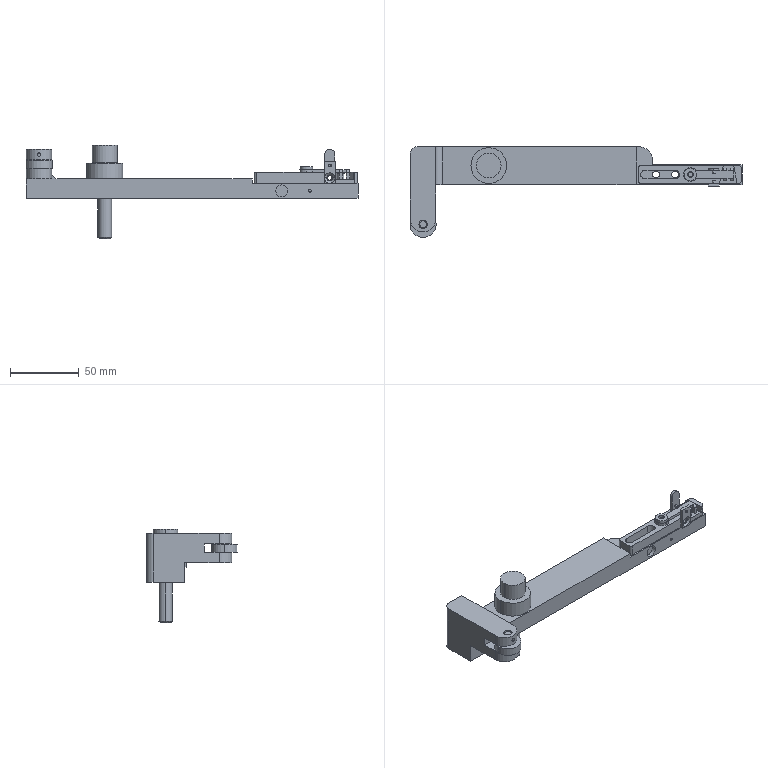Assembly | SolidWorks | mm | 13 component files | 13 solids | 202 faces | box 241.25 x 66 x 68 mm | volume 117753 mm3 | plane 98 | cylinder 82 | cone 22 | commonest cylinder face diameters 2 x10 5 x10 6 x8 4 x8 10 x7 8 x4 16 x4 12 x4
Bill of materials:
Bearing626z | 1 |  | Thick flat annular disc (ring) with a central through-hole; plain cylindrical outer face and flat parallel faces.
BSH3-02-05SmallWheel | 1 |  | Short solid cylinder, about as long as it is wide, with a chamfer on both end edges.
BSH3-02-06SpringRetainer | 1 |  | Rectangular flat plate with a small round through-hole near one end and a larger through-hole near the other end that has a conical countersink on one face.
BSH3-02-07Pin | 2 |  | Solid cylindrical pin, roughly twice as long as its diameter, with a chamfer on both ends.
BSH3-02-08BendingPlate | 1 |  | Flat bar-like bent part: an elongated strip ending in a ring-shaped eye with a round hole at one end; an upright tab with a rounded top and a small hole rising from the strip; and at the other end, legs/tabs bent down to form a U-shaped or channel-like clip section.
BSH3-02-09Gasket | 1 |  | Flanged bushing: a larger-diameter cylindrical flange plus a smaller-diameter cylindrical spigot on one side, with a straight central through-bore.
BSH3-02-10FeedBlock2 | 1 |  | Elongated rectangular bar with rounded corners. It has a long through slot with rounded ends, a small vertical through-hole, a cross hole through the side, and a stepped end region with a notch/slot cut across it.
BSH3-03-01Lever | 1 |  | Long arm/lever-like bar. At one end is a forked clevis with two parallel lugs, each with a small hole. Partway along is a raised cylindrical boss with a large bore. The far end is a narrower, stepped-down section with several small holes.
BSH3-03-02RotatingPin | 1 |  | Slender solid cylindrical pin, several diameters long, with a small chamfer on both ends.
BSH3-03-08CopperRing | 1 |  | Thin-walled cylindrical tube/sleeve with a straight through-bore and plain square-cut ends.
BSH3-03-39Pin | 1 |  | Short solid cylinder, a little longer than its diameter. One end is clearly chamfered; the other end looks square or has a much smaller edge break.
ScrewM10 | 1 |  | Stepped solid cylindrical pin with three diameters: a larger short head, a middle shank, and a slightly smaller end shank with a small chamfer at the tip.
Mates:
1. concentric | BSH3-03-01Lever-1 face at (-60.871, 27.262, -25.939) dir (0, 0, 1) r 8 | BSH3-03-08CopperRing-1 face at (-60.871, 27.262, 0.0608) dir (0, 0, -1) r 8
2. coincident | BSH3-03-01Lever-1 face at (-117.871, 41.012, -25.939) dir (0, 0, -1) | BSH3-03-08CopperRing-1 face at (-60.871, 27.262, -25.939) dir (0, 0, -1)
3. parallel | BSH3-03-01Lever-1 plane at (-117.871, 13.512, -25.939) dir (0, 1, 0) | BSH3-03-08CopperRing-1 plane at (-60.871, 27.262, -25.939) dir (0, 1, 0)
4. concentric | BSH3-03-01Lever-1 face at (-108.621, -15.488, -25.939) dir (0, 0, 1) r 3 | BSH3-03-02RotatingPin-1 face at (-108.621, -15.488, 8.561) dir (0, 0, -1) r 3
5. distance | BSH3-03-01Lever-1 face at (-108.621, -11.738, 9.561) dir (0, 0, 1) | BSH3-03-02RotatingPin-1 face at (-108.621, -15.488, 8.561) dir (0, 0, 1)
6. parallel | BSH3-03-01Lever-1 face at (-117.871, 13.512, -11.939) dir (0, -1, 0) | BSH3-03-02RotatingPin-1 plane at (-108.621, -15.488, -11.439) dir (0, 1, 0)
7. concentric | BSH3-03-02RotatingPin-1 face at (-108.621, -15.488, 8.561) dir (0, 0, -1) r 3 | Bearing626z-1 face at (-108.621, -15.488, 1.811) dir (0, 0, -1) r 9.5
8. distance | Bearing626z-1 face at (-108.621, -15.488, 1.811) dir (0, 0, 1) | BSH3-03-01Lever-1 face at (123.129, -0.9884, 1.861) dir (0, 0, -1)
9. parallel | BSH3-03-01Lever-1 face at (-117.871, 13.512, -11.939) dir (0, -1, 0) | Bearing626z-1 plane at (-108.621, -15.488, -4.189) dir (0, -1, 0)
10. concentric | ScrewM10-1 face at (-60.871, 27.262, -55.439) dir (0, 0, -1) r 6 | BSH3-03-08CopperRing-1 face at (-60.871, 27.262, 0.0608) dir (0, 0, -1) r 6
11. coincident | BSH3-03-08CopperRing-1 face at (-60.871, 27.262, 0.0608) dir (0, 0, 1) | ScrewM10-1 face at (-51.871, 27.262, 0.0608) dir (0, 0, -1)
12. parallel | BSH3-03-01Lever-1 face at (-117.871, 13.512, -11.939) dir (0, -1, 0) | ScrewM10-1 plane at (-60.871, 27.262, 12.561) dir (0, 1, 0)
13. coincident | BSH3-03-01Lever-1 face at (123.129, 41.012, -15.239) dir (0, 0, 1) | BSH3-02-00ARubberBlankingAssembly2-1/BSH3-02-10FeedBlock2-1 face at (47.629, 27.262, -15.239) dir (0, 0, -1)
14. parallel | BSH3-03-01Lever-1 face at (123.129, 28.012, -11.939) dir (0, 1, 0) | BSH3-02-00ARubberBlankingAssembly2-1/BSH3-02-10FeedBlock2-1 face at (122.629, 27.262, -7.239) dir (0, 1, 0)
15. concentric | BSH3-03-01Lever-1 face at (74.629, 20.762, -15.239) dir (0, 0, 1) r 2.5 | BSH3-02-00ARubberBlankingAssembly2-1/BSH3-02-10FeedBlock2-1 face at (74.629, 20.762, -7.239) dir (0, 0, -1) r 3.1
16. coincident | BSH3-03-01Lever-1 face at (88.129, 18.012, -20.589) dir (0, 1, 0) | BSH3-03-39Pin-1 face at (88.129, 18.012, -20.589) dir (0, -1, 0)
17. concentric | BSH3-03-01Lever-1 face at (88.129, 18.012, -20.589) dir (0, 1, 0) r 4 | BSH3-03-39Pin-1 face at (88.129, 28.012, -20.589) dir (0, -1, 0) r 4
18. coincident | BSH3-02-10FeedBlock2-1 face at (-14.378, -37.036, 7.842) dir (-1, 0, 0) | BSH3-02-06SpringRetainer-1 face at (-14.378, -13.036, -0.1581) dir (1, 0, 0)
19. concentric | BSH3-02-10FeedBlock2-1 face at (-14.378, -17.036, 3.842) dir (-1, 0, 0) r 1.65 | BSH3-02-06SpringRetainer-1 face at (-16.378, -17.036, 3.842) dir (1, 0, 0) r 2.25
20. parallel | BSH3-02-06SpringRetainer-1 face at (-16.378, -21.036, -0.1581) dir (0, 0, -1) | BSH3-02-10FeedBlock2-1 face at (-1.378, 37.964, -0.1581) dir (0, 0, -1)
21. coincident | BSH3-02-10FeedBlock2-1 face at (-1.378, 37.964, 7.842) dir (0, 0, 1) | BSH3-02-09Gasket-1 face at (-5.828, -0.03595, 7.842) dir (0, 0, -1)
22. concentric | BSH3-02-10FeedBlock2-1 face at (-7.878, -0.03595, 7.842) dir (0, 0, 1) r 1.65 | BSH3-02-09Gasket-1 face at (-7.878, -0.03595, 11.942) dir (0, 0, 1) r 4.5
23. parallel | BSH3-02-10FeedBlock2-1 face at (-14.378, 37.964, 7.842) dir (0, 1, 0) | BSH3-02-09Gasket-1 plane at (-7.878, -0.03595, 11.942) dir (0, 1, 0)
24. coincident | BSH3-02-08BendingPlate-1 face at (-7.878, -0.03595, 7.842) dir (0, 0, -1) | BSH3-02-10FeedBlock2-1 face at (-1.378, 37.964, 7.842) dir (0, 0, 1)
25. concentric | BSH3-02-09Gasket-1 face at (-7.878, -0.03595, 11.942) dir (0, 0, 1) r 2.05 | BSH3-02-08BendingPlate-1 face at (-7.878, -0.03595, 7.842) dir (0, 0, 1) r 2.5
26. parallel | BSH3-02-10FeedBlock2-1 face at (-1.378, -37.036, 7.842) dir (1, 0, 0) | BSH3-02-08BendingPlate-1 face at (-3.228, -17.036, 21.342) dir (1, 0, 0)
27. coincident | BSH3-02-10FeedBlock2-1 face at (-14.378, -34.036, 2.542) dir (0, 0, 1) | BSH3-02-05SmallWheel-1 face at (-7.878, -25.102, 2.542) dir (0, 0, -1)
28. distance | BSH3-02-05SmallWheel-1 plane at (-7.878, -25.102, 2.542) dir (1, 0, 0) | BSH3-02-10FeedBlock2-1 face at (-1.378, -37.036, 7.842) dir (1, 0, 0)
29. concentric | BSH3-02-06SpringRetainer-1 face at (-16.378, -17.036, 12.842) dir (1, 0, 0) r 1 | BSH3-02-07Pin-1 face at (-12.378, -17.036, 12.842) dir (-1, 0, 0) r 1
30. coincident | BSH3-02-06SpringRetainer-1 face at (-16.378, -13.036, -0.1581) dir (-1, 0, 0) | BSH3-02-07Pin-1 face at (-16.378, -17.036, 12.842) dir (-1, 0, 0)
31. parallel | BSH3-02-06SpringRetainer-1 face at (-16.378, -21.036, 15.842) dir (0, 0, 1) | BSH3-02-07Pin-1 plane at (-16.378, -17.036, 12.842) dir (0, 0, -1)
32. tangent | BSH3-02-07Pin-2 face at (-3.228, -17.036, 12.342) dir (-1, 0, 0) r 1 | BSH3-02-08BendingPlate-1 face at (-3.228, -17.036, 12.342) dir (-1, 0, 0) r 1
33. coincident | BSH3-02-08BendingPlate-1 face at (-3.228, -17.036, 21.342) dir (1, 0, 0) | BSH3-02-07Pin-2 face at (-3.228, -17.036, 12.342) dir (1, 0, 0)
34. parallel | BSH3-02-10FeedBlock2-1 face at (-1.378, 37.964, 7.842) dir (0, 0, 1) | BSH3-02-07Pin-1 plane at (-16.378, -17.036, 12.842) dir (0, 0, -1)